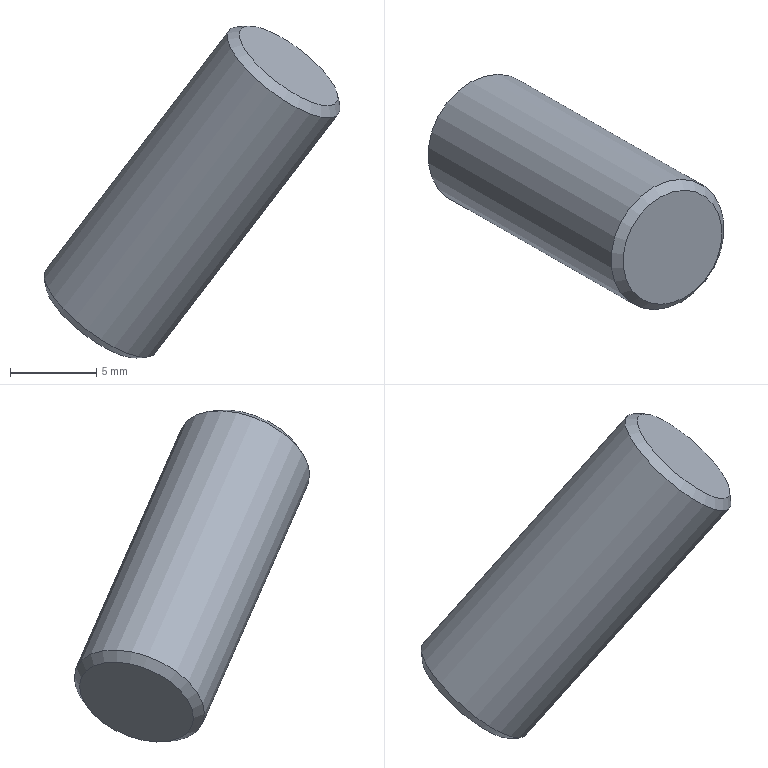Component | NX | XUAN_ZHUAN_ZHOU | 1 solid | 5 faces | box 17.16 x 13.66 x 19.25 mm | volume 974 mm3 | plane 2 | cone 2 | cylinder 1 | commonest cylinder face diameters 8 x1
STEP:
#1=CARTESIAN_POINT('',(0.,0.,0.));
#2=DIRECTION('',(0.,0.,1.));
#3=DIRECTION('',(1.,0.,0.));
#4=AXIS2_PLACEMENT_3D('',#1,#2,#3);
#5=CARTESIAN_POINT('',(-81.621,-76.17,-44.444));
#6=VERTEX_POINT('',#5);
#7=CARTESIAN_POINT('',(-81.621,-72.509,-42.832));
#8=DIRECTION('',(0.5736,-0.3301,0.7497));
#9=DIRECTION('',(0.,-0.9152,-0.4029));
#10=AXIS2_PLACEMENT_3D('',#7,#8,#9);
#11=CIRCLE('',#10,4.);
#12=CARTESIAN_POINT('',(-70.723,-78.78,-28.587));
#13=DIRECTION('',(-0.5736,0.3301,-0.7497));
#14=DIRECTION('',(0.,0.9152,0.4029));
#15=AXIS2_PLACEMENT_3D('',#12,#13,#14);
#16=CYLINDRICAL_SURFACE('',#15,4.);
#17=CARTESIAN_POINT('',(9.425,19.));
#18=DIRECTION('',(-1.,0.));
#19=VECTOR('',#18,1.);
#20=LINE('',#17,#19);
#21=(GEOMETRIC_REPRESENTATION_CONTEXT(2)PARAMETRIC_REPRESENTATION_CONTEXT()REPRESENTATION_CONTEXT('',''));
#22=DEFINITIONAL_REPRESENTATION('',(#20),#21);
#23=PCURVE('',#16,#22);
#24=CARTESIAN_POINT('',(-81.621,-72.509,-42.832));
#25=DIRECTION('',(0.5736,-0.3301,0.7497));
#26=DIRECTION('',(0.,-0.9152,-0.4029));
#27=AXIS2_PLACEMENT_3D('',#24,#25,#26);
#28=CONICAL_SURFACE('',#27,4.,0.7854);
#29=CARTESIAN_POINT('',(0.,-0.));
#30=DIRECTION('',(1.,0.));
#31=VECTOR('',#30,1.);
#32=LINE('',#29,#31);
#33=(GEOMETRIC_REPRESENTATION_CONTEXT(2)PARAMETRIC_REPRESENTATION_CONTEXT()REPRESENTATION_CONTEXT('',''));
#34=DEFINITIONAL_REPRESENTATION('',(#32),#33);
#35=PCURVE('',#28,#34);
#36=SURFACE_CURVE('',#11,(#23,#35),.PCURVE_S1.);
#37=EDGE_CURVE('',#6,#6,#36,.T.);
#38=ORIENTED_EDGE('',*,*,#37,.T.);
#39=CARTESIAN_POINT('',(-71.01,-82.276,-30.574));
#40=VERTEX_POINT('',#39);
#41=CARTESIAN_POINT('',(-71.01,-82.276,-30.574));
#42=CARTESIAN_POINT('',(-81.621,-76.17,-44.444));
#43=B_SPLINE_CURVE_WITH_KNOTS('',1,(#41,#42),.UNSPECIFIED.,.F.,.F.,(2,2),(0.5,19.),.PIECEWISE_BEZIER_KNOTS.);
#44=CARTESIAN_POINT('',(3.142,0.));
#45=DIRECTION('',(0.,1.));
#46=VECTOR('',#45,1.);
#47=LINE('',#44,#46);
#48=(GEOMETRIC_REPRESENTATION_CONTEXT(2)PARAMETRIC_REPRESENTATION_CONTEXT()REPRESENTATION_CONTEXT('',''));
#49=DEFINITIONAL_REPRESENTATION('',(#47),#48);
#50=PCURVE('',#16,#49);
#51=CARTESIAN_POINT('',(9.425,0.));
#52=DIRECTION('',(0.,1.));
#53=VECTOR('',#52,1.);
#54=LINE('',#51,#53);
#55=(GEOMETRIC_REPRESENTATION_CONTEXT(2)PARAMETRIC_REPRESENTATION_CONTEXT()REPRESENTATION_CONTEXT('',''));
#56=DEFINITIONAL_REPRESENTATION('',(#54),#55);
#57=PCURVE('',#16,#56);
#58=SEAM_CURVE('',#43,(#50,#57),.PCURVE_S1.);
#59=EDGE_CURVE('',#40,#6,#58,.T.);
#60=ORIENTED_EDGE('',*,*,#59,.F.);
#61=CARTESIAN_POINT('',(-71.01,-78.615,-28.962));
#62=DIRECTION('',(-0.5736,0.3301,-0.7497));
#63=DIRECTION('',(-0.,-0.9152,-0.4029));
#64=AXIS2_PLACEMENT_3D('',#61,#62,#63);
#65=CIRCLE('',#64,4.);
#66=CARTESIAN_POINT('',(3.142,0.5));
#67=DIRECTION('',(1.,0.));
#68=VECTOR('',#67,1.);
#69=LINE('',#66,#68);
#70=(GEOMETRIC_REPRESENTATION_CONTEXT(2)PARAMETRIC_REPRESENTATION_CONTEXT()REPRESENTATION_CONTEXT('',''));
#71=DEFINITIONAL_REPRESENTATION('',(#69),#70);
#72=PCURVE('',#16,#71);
#73=CARTESIAN_POINT('',(-70.723,-78.78,-28.587));
#74=DIRECTION('',(-0.5736,0.3301,-0.7497));
#75=DIRECTION('',(-0.,0.9152,0.4029));
#76=AXIS2_PLACEMENT_3D('',#73,#74,#75);
#77=CONICAL_SURFACE('',#76,3.5,0.7854);
#78=CARTESIAN_POINT('',(3.142,0.5));
#79=DIRECTION('',(1.,0.));
#80=VECTOR('',#79,1.);
#81=LINE('',#78,#80);
#82=(GEOMETRIC_REPRESENTATION_CONTEXT(2)PARAMETRIC_REPRESENTATION_CONTEXT()REPRESENTATION_CONTEXT('',''));
#83=DEFINITIONAL_REPRESENTATION('',(#81),#82);
#84=PCURVE('',#77,#83);
#85=SURFACE_CURVE('',#65,(#72,#84),.PCURVE_S1.);
#86=EDGE_CURVE('',#40,#40,#85,.T.);
#87=ORIENTED_EDGE('',*,*,#86,.T.);
#88=ORIENTED_EDGE('',*,*,#59,.T.);
#89=EDGE_LOOP('',(#38,#60,#87,#88));
#90=FACE_BOUND('',#89,.T.);
#91=ADVANCED_FACE('',(#90),#16,.T.);
#92=CARTESIAN_POINT('',(-70.723,-81.983,-29.998));
#93=VERTEX_POINT('',#92);
#94=CARTESIAN_POINT('',(-70.723,-78.78,-28.587));
#95=DIRECTION('',(0.5736,-0.3301,0.7497));
#96=DIRECTION('',(-0.,-0.9152,-0.4029));
#97=AXIS2_PLACEMENT_3D('',#94,#95,#96);
#98=CIRCLE('',#97,3.5);
#99=CARTESIAN_POINT('',(-70.723,-78.78,-28.587));
#100=DIRECTION('',(0.5736,-0.3301,0.7497));
#101=DIRECTION('',(0.,-0.9152,-0.4029));
#102=AXIS2_PLACEMENT_3D('',#99,#100,#101);
#103=PLANE('',#102);
#104=CARTESIAN_POINT('',(0.,0.));
#105=DIRECTION('',(1.,-0.));
#106=AXIS2_PLACEMENT_2D('',#104,#105);
#107=CIRCLE('',#106,3.5);
#108=(GEOMETRIC_REPRESENTATION_CONTEXT(2)PARAMETRIC_REPRESENTATION_CONTEXT()REPRESENTATION_CONTEXT('',''));
#109=DEFINITIONAL_REPRESENTATION('',(#107),#108);
#110=PCURVE('',#103,#109);
#111=CARTESIAN_POINT('',(9.425,0.));
#112=DIRECTION('',(-1.,0.));
#113=VECTOR('',#112,1.);
#114=LINE('',#111,#113);
#115=(GEOMETRIC_REPRESENTATION_CONTEXT(2)PARAMETRIC_REPRESENTATION_CONTEXT()REPRESENTATION_CONTEXT('',''));
#116=DEFINITIONAL_REPRESENTATION('',(#114),#115);
#117=PCURVE('',#77,#116);
#118=SURFACE_CURVE('',#98,(#110,#117),.PCURVE_S1.);
#119=EDGE_CURVE('',#93,#93,#118,.T.);
#120=ORIENTED_EDGE('',*,*,#119,.T.);
#121=EDGE_LOOP('',(#120));
#122=FACE_BOUND('',#121,.T.);
#123=ADVANCED_FACE('',(#122),#103,.T.);
#124=CARTESIAN_POINT('',(-81.908,-75.547,-44.617));
#125=VERTEX_POINT('',#124);
#126=CARTESIAN_POINT('',(-81.908,-72.344,-43.207));
#127=DIRECTION('',(-0.5736,0.3301,-0.7497));
#128=DIRECTION('',(-0.,-0.9152,-0.4029));
#129=AXIS2_PLACEMENT_3D('',#126,#127,#128);
#130=CIRCLE('',#129,3.5);
#131=CARTESIAN_POINT('',(-81.908,-72.344,-43.207));
#132=DIRECTION('',(0.5736,-0.3301,0.7497));
#133=DIRECTION('',(0.,-0.9152,-0.4029));
#134=AXIS2_PLACEMENT_3D('',#131,#132,#133);
#135=PLANE('',#134);
#136=CARTESIAN_POINT('',(3.5,-0.));
#137=CARTESIAN_POINT('',(3.5,-6.062));
#138=CARTESIAN_POINT('',(-1.75,-3.031));
#139=CARTESIAN_POINT('',(-7.,0.));
#140=CARTESIAN_POINT('',(-1.75,3.031));
#141=CARTESIAN_POINT('',(3.5,6.062));
#142=CARTESIAN_POINT('',(3.5,-0.));
#143=(BOUNDED_CURVE()B_SPLINE_CURVE(2,(#136,#137,#138,#139,#140,#141,#142),.UNSPECIFIED.,.T.,.F.)B_SPLINE_CURVE_WITH_KNOTS((1,2,2,2,2,1),(-2.094,0.,2.094,4.189,6.283,8.378),.UNSPECIFIED.)CURVE()GEOMETRIC_REPRESENTATION_ITEM()RATIONAL_B_SPLINE_CURVE((1.,0.5,1.,0.5,1.,0.5,1.))REPRESENTATION_ITEM(''));
#144=(GEOMETRIC_REPRESENTATION_CONTEXT(2)PARAMETRIC_REPRESENTATION_CONTEXT()REPRESENTATION_CONTEXT('',''));
#145=DEFINITIONAL_REPRESENTATION('',(#143),#144);
#146=PCURVE('',#135,#145);
#147=CARTESIAN_POINT('',(6.283,-0.5));
#148=DIRECTION('',(-1.,0.));
#149=VECTOR('',#148,1.);
#150=LINE('',#147,#149);
#151=(GEOMETRIC_REPRESENTATION_CONTEXT(2)PARAMETRIC_REPRESENTATION_CONTEXT()REPRESENTATION_CONTEXT('',''));
#152=DEFINITIONAL_REPRESENTATION('',(#150),#151);
#153=PCURVE('',#28,#152);
#154=SURFACE_CURVE('',#130,(#146,#153),.PCURVE_S1.);
#155=EDGE_CURVE('',#125,#125,#154,.T.);
#156=ORIENTED_EDGE('',*,*,#155,.T.);
#157=EDGE_LOOP('',(#156));
#158=FACE_BOUND('',#157,.T.);
#159=ADVANCED_FACE('',(#158),#135,.F.);
#160=ORIENTED_EDGE('',*,*,#86,.F.);
#161=CARTESIAN_POINT('',(-70.723,-81.983,-29.998));
#162=CARTESIAN_POINT('',(-71.01,-82.276,-30.574));
#163=B_SPLINE_CURVE_WITH_KNOTS('',1,(#161,#162),.UNSPECIFIED.,.F.,.F.,(2,2),(0.,0.7071),.PIECEWISE_BEZIER_KNOTS.);
#164=CARTESIAN_POINT('',(3.142,0.));
#165=DIRECTION('',(0.,1.));
#166=VECTOR('',#165,1.);
#167=LINE('',#164,#166);
#168=(GEOMETRIC_REPRESENTATION_CONTEXT(2)PARAMETRIC_REPRESENTATION_CONTEXT()REPRESENTATION_CONTEXT('',''));
#169=DEFINITIONAL_REPRESENTATION('',(#167),#168);
#170=PCURVE('',#77,#169);
#171=CARTESIAN_POINT('',(9.425,0.));
#172=DIRECTION('',(0.,1.));
#173=VECTOR('',#172,1.);
#174=LINE('',#171,#173);
#175=(GEOMETRIC_REPRESENTATION_CONTEXT(2)PARAMETRIC_REPRESENTATION_CONTEXT()REPRESENTATION_CONTEXT('',''));
#176=DEFINITIONAL_REPRESENTATION('',(#174),#175);
#177=PCURVE('',#77,#176);
#178=SEAM_CURVE('',#163,(#170,#177),.PCURVE_S1.);
#179=EDGE_CURVE('',#93,#40,#178,.T.);
#180=ORIENTED_EDGE('',*,*,#179,.F.);
#181=ORIENTED_EDGE('',*,*,#119,.F.);
#182=ORIENTED_EDGE('',*,*,#179,.T.);
#183=EDGE_LOOP('',(#160,#180,#181,#182));
#184=FACE_BOUND('',#183,.T.);
#185=ADVANCED_FACE('',(#184),#77,.T.);
#186=ORIENTED_EDGE('',*,*,#155,.F.);
#187=CARTESIAN_POINT('',(-81.908,-75.547,-44.617));
#188=CARTESIAN_POINT('',(-81.621,-76.17,-44.444));
#189=B_SPLINE_CURVE_WITH_KNOTS('',1,(#187,#188),.UNSPECIFIED.,.F.,.F.,(2,2),(-0.7071,0.),.PIECEWISE_BEZIER_KNOTS.);
#190=CARTESIAN_POINT('',(6.283,0.));
#191=DIRECTION('',(0.,1.));
#192=VECTOR('',#191,1.);
#193=LINE('',#190,#192);
#194=(GEOMETRIC_REPRESENTATION_CONTEXT(2)PARAMETRIC_REPRESENTATION_CONTEXT()REPRESENTATION_CONTEXT('',''));
#195=DEFINITIONAL_REPRESENTATION('',(#193),#194);
#196=PCURVE('',#28,#195);
#197=CARTESIAN_POINT('',(0.,0.));
#198=DIRECTION('',(0.,1.));
#199=VECTOR('',#198,1.);
#200=LINE('',#197,#199);
#201=(GEOMETRIC_REPRESENTATION_CONTEXT(2)PARAMETRIC_REPRESENTATION_CONTEXT()REPRESENTATION_CONTEXT('',''));
#202=DEFINITIONAL_REPRESENTATION('',(#200),#201);
#203=PCURVE('',#28,#202);
#204=SEAM_CURVE('',#189,(#196,#203),.PCURVE_S1.);
#205=EDGE_CURVE('',#125,#6,#204,.T.);
#206=ORIENTED_EDGE('',*,*,#205,.T.);
#207=ORIENTED_EDGE('',*,*,#37,.F.);
#208=ORIENTED_EDGE('',*,*,#205,.F.);
#209=EDGE_LOOP('',(#186,#206,#207,#208));
#210=FACE_BOUND('',#209,.T.);
#211=ADVANCED_FACE('',(#210),#28,.T.);
#212=CLOSED_SHELL('',(#91,#123,#159,#185,#211));
#213=MANIFOLD_SOLID_BREP('',#212);
#214=(LENGTH_UNIT()NAMED_UNIT(*)SI_UNIT(.MILLI.,.METRE.));
#215=UNCERTAINTY_MEASURE_WITH_UNIT(LENGTH_MEASURE(0.00001),#214,'','');
#216=(NAMED_UNIT(*)PLANE_ANGLE_UNIT()SI_UNIT($,.RADIAN.));
#217=(NAMED_UNIT(*)SI_UNIT($,.STERADIAN.)SOLID_ANGLE_UNIT());
#218=(GEOMETRIC_REPRESENTATION_CONTEXT(3)GLOBAL_UNCERTAINTY_ASSIGNED_CONTEXT((#215))GLOBAL_UNIT_ASSIGNED_CONTEXT((#214,#216,#217))REPRESENTATION_CONTEXT('',''));
#219=ADVANCED_BREP_SHAPE_REPRESENTATION('',(#4,#213),#218);